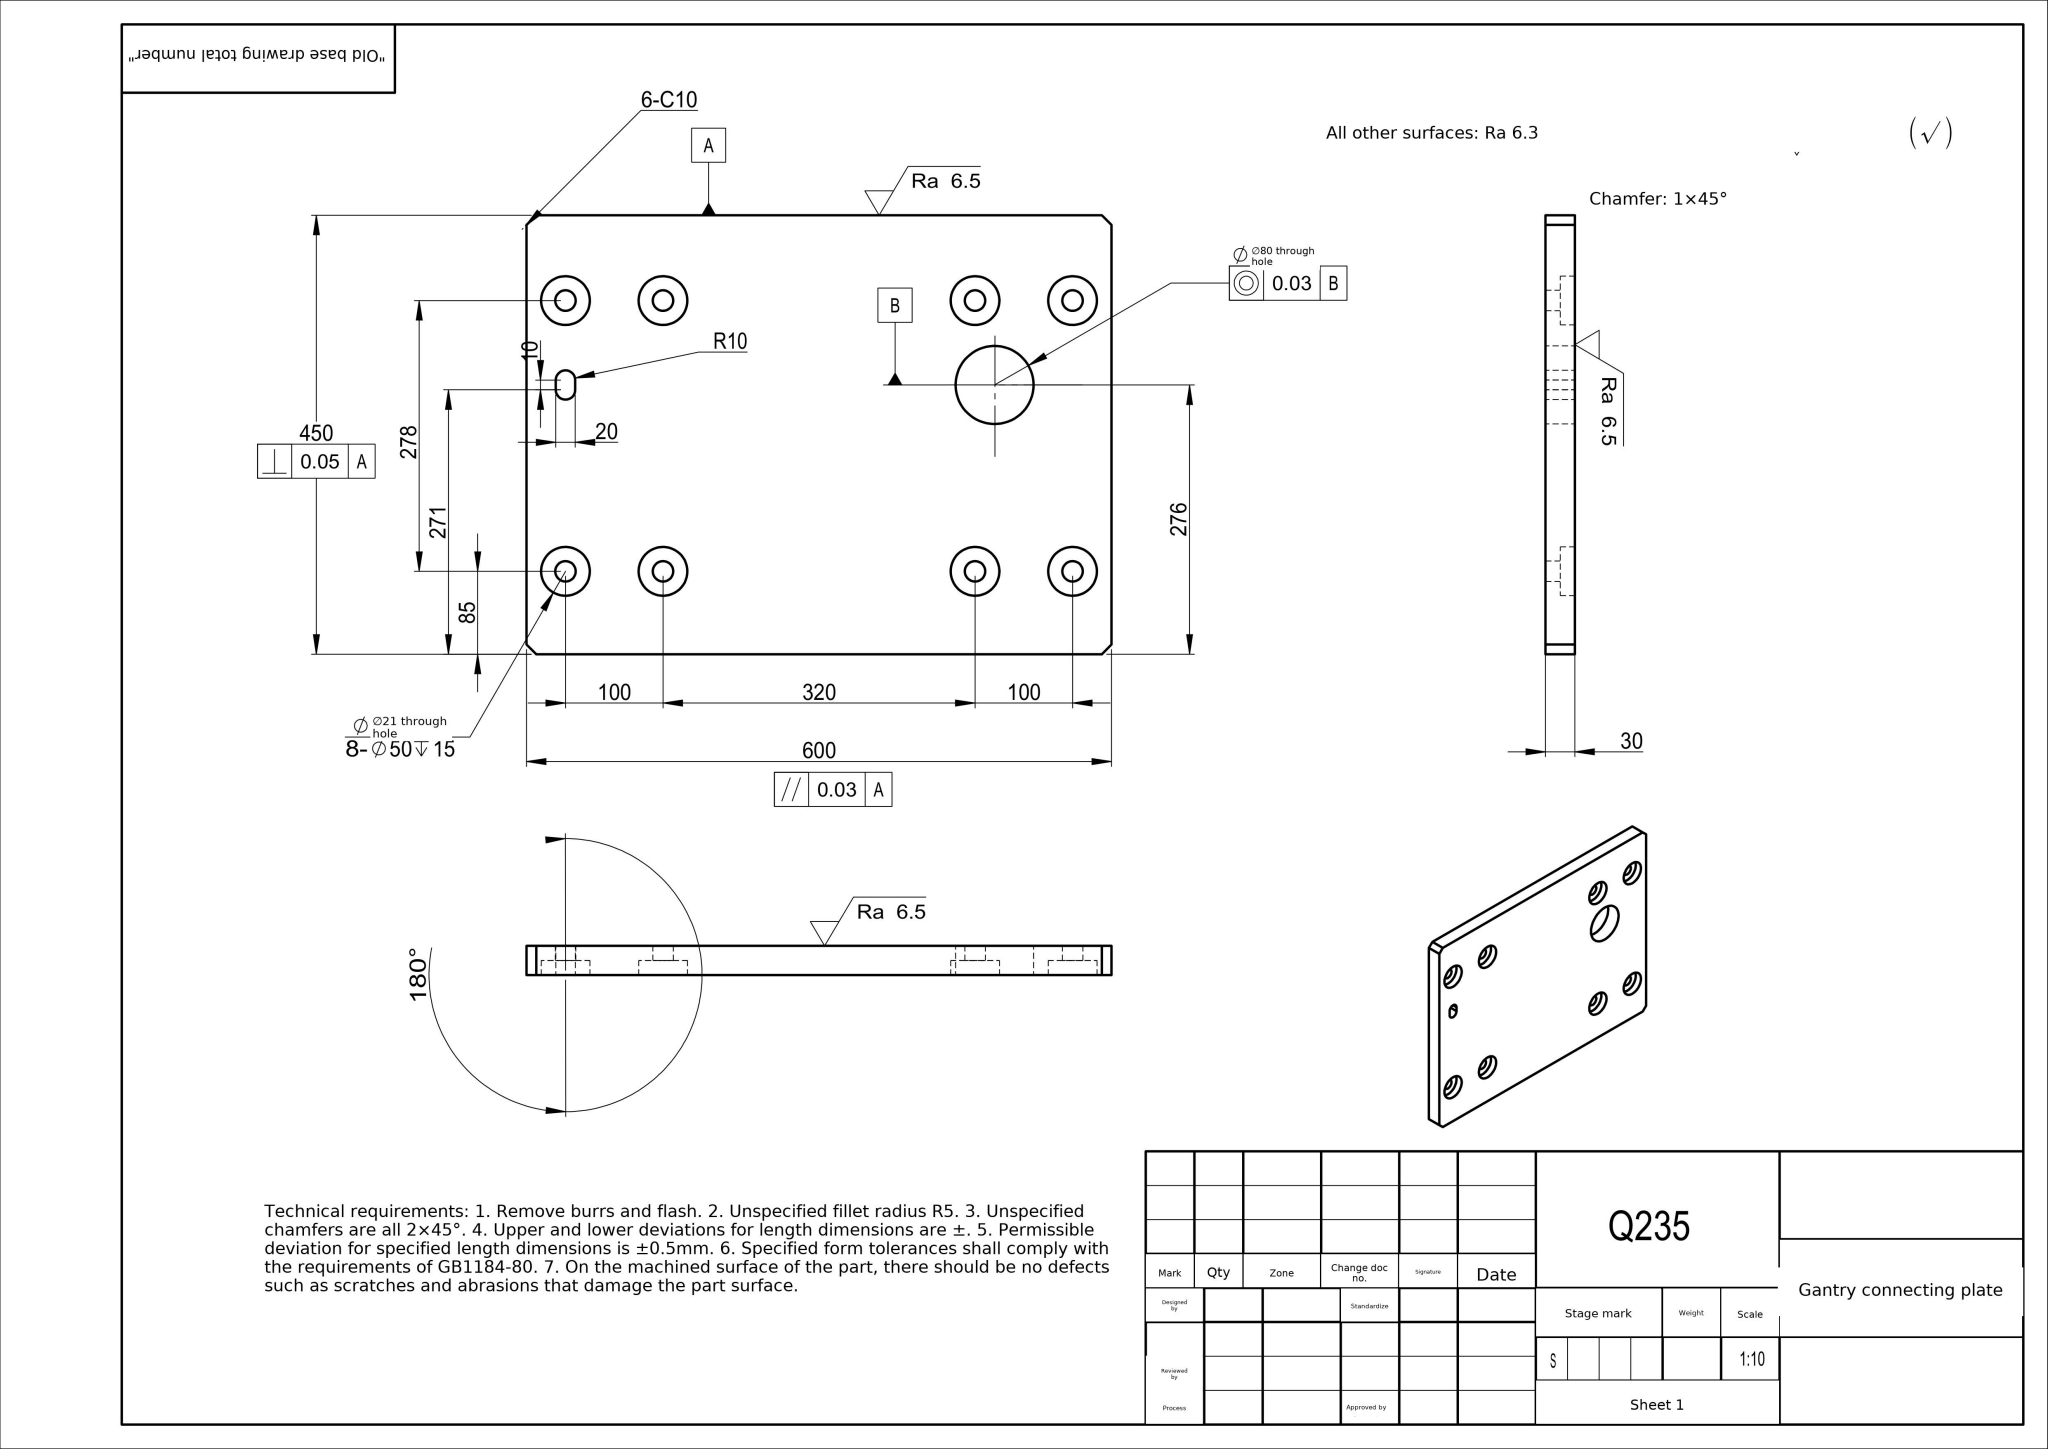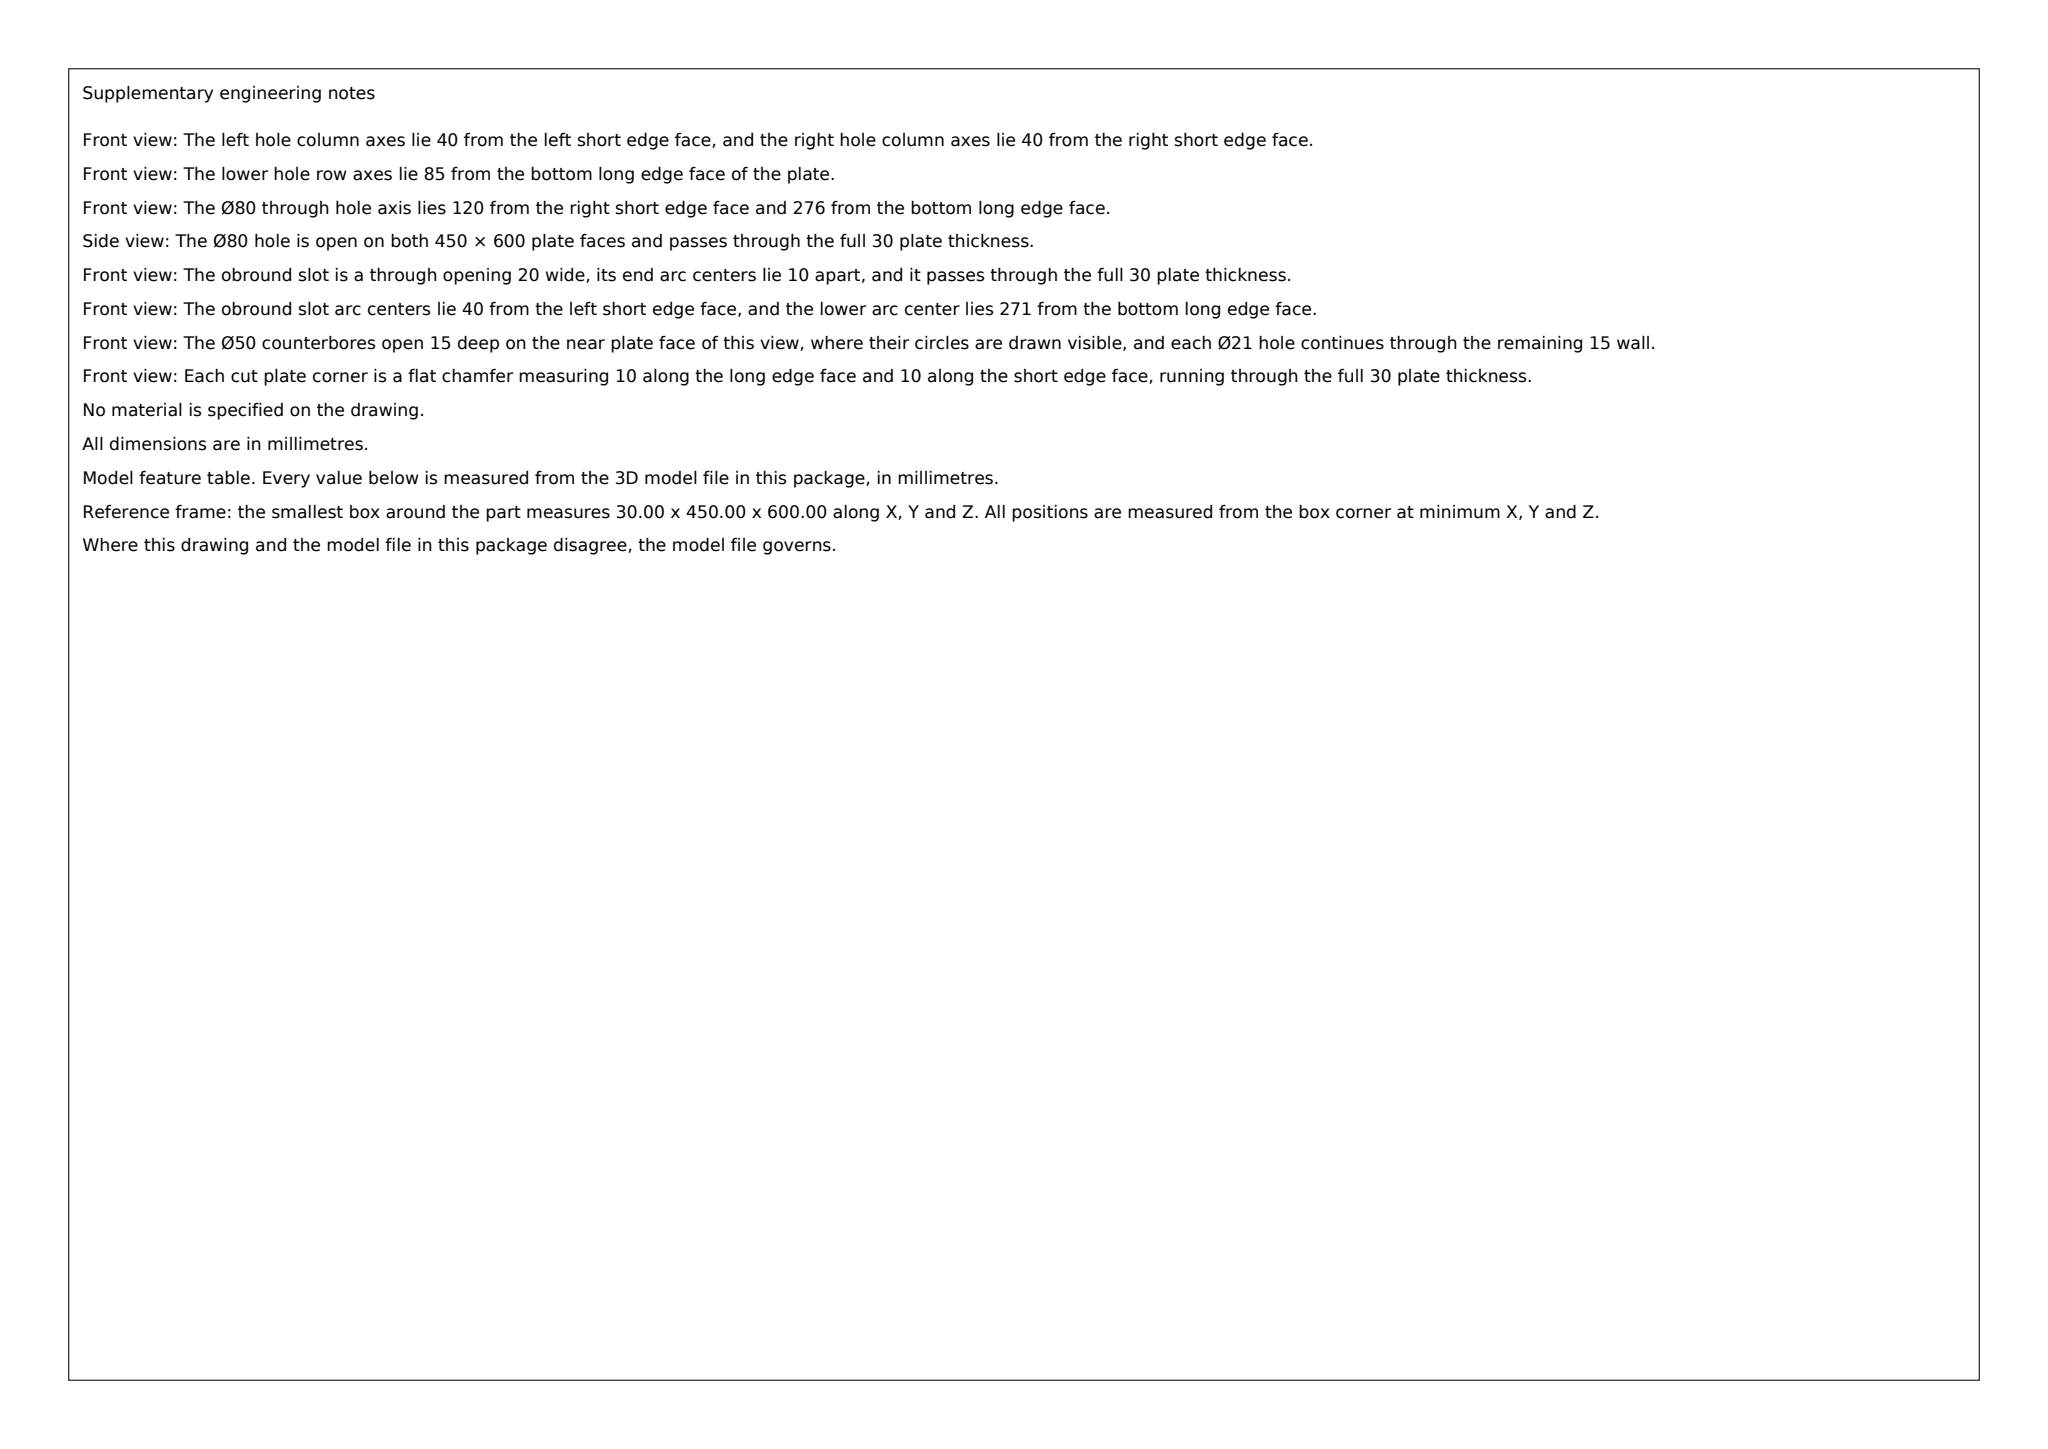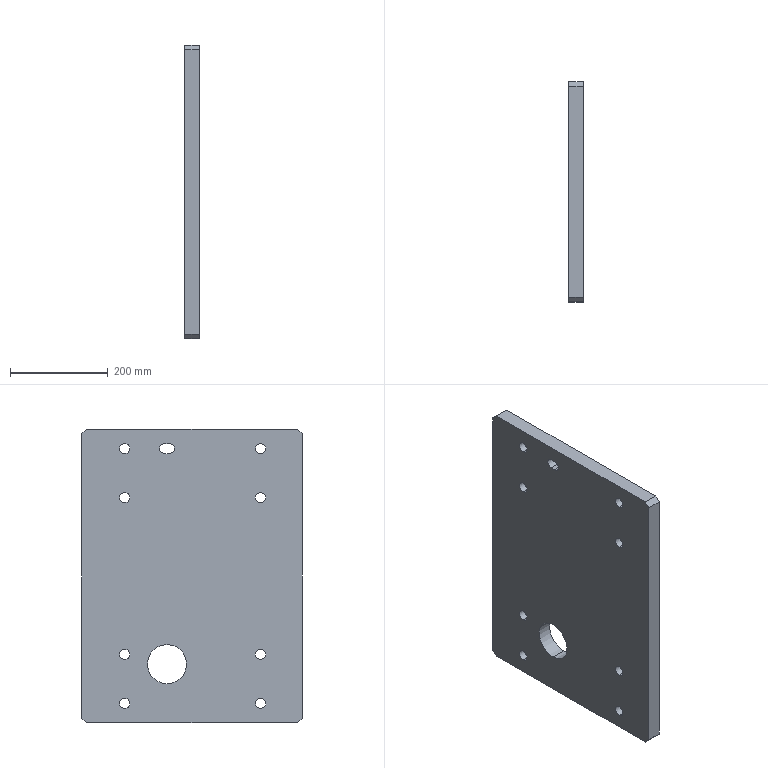Part | SolidWorks | mm | 1 solid | 56 faces | box 30 x 450 x 600 mm | volume 7650596 mm3 | cylinder 36 | plane 20 | commonest cylinder face diameters 21 x16 50 x16 80 x2 20 x2